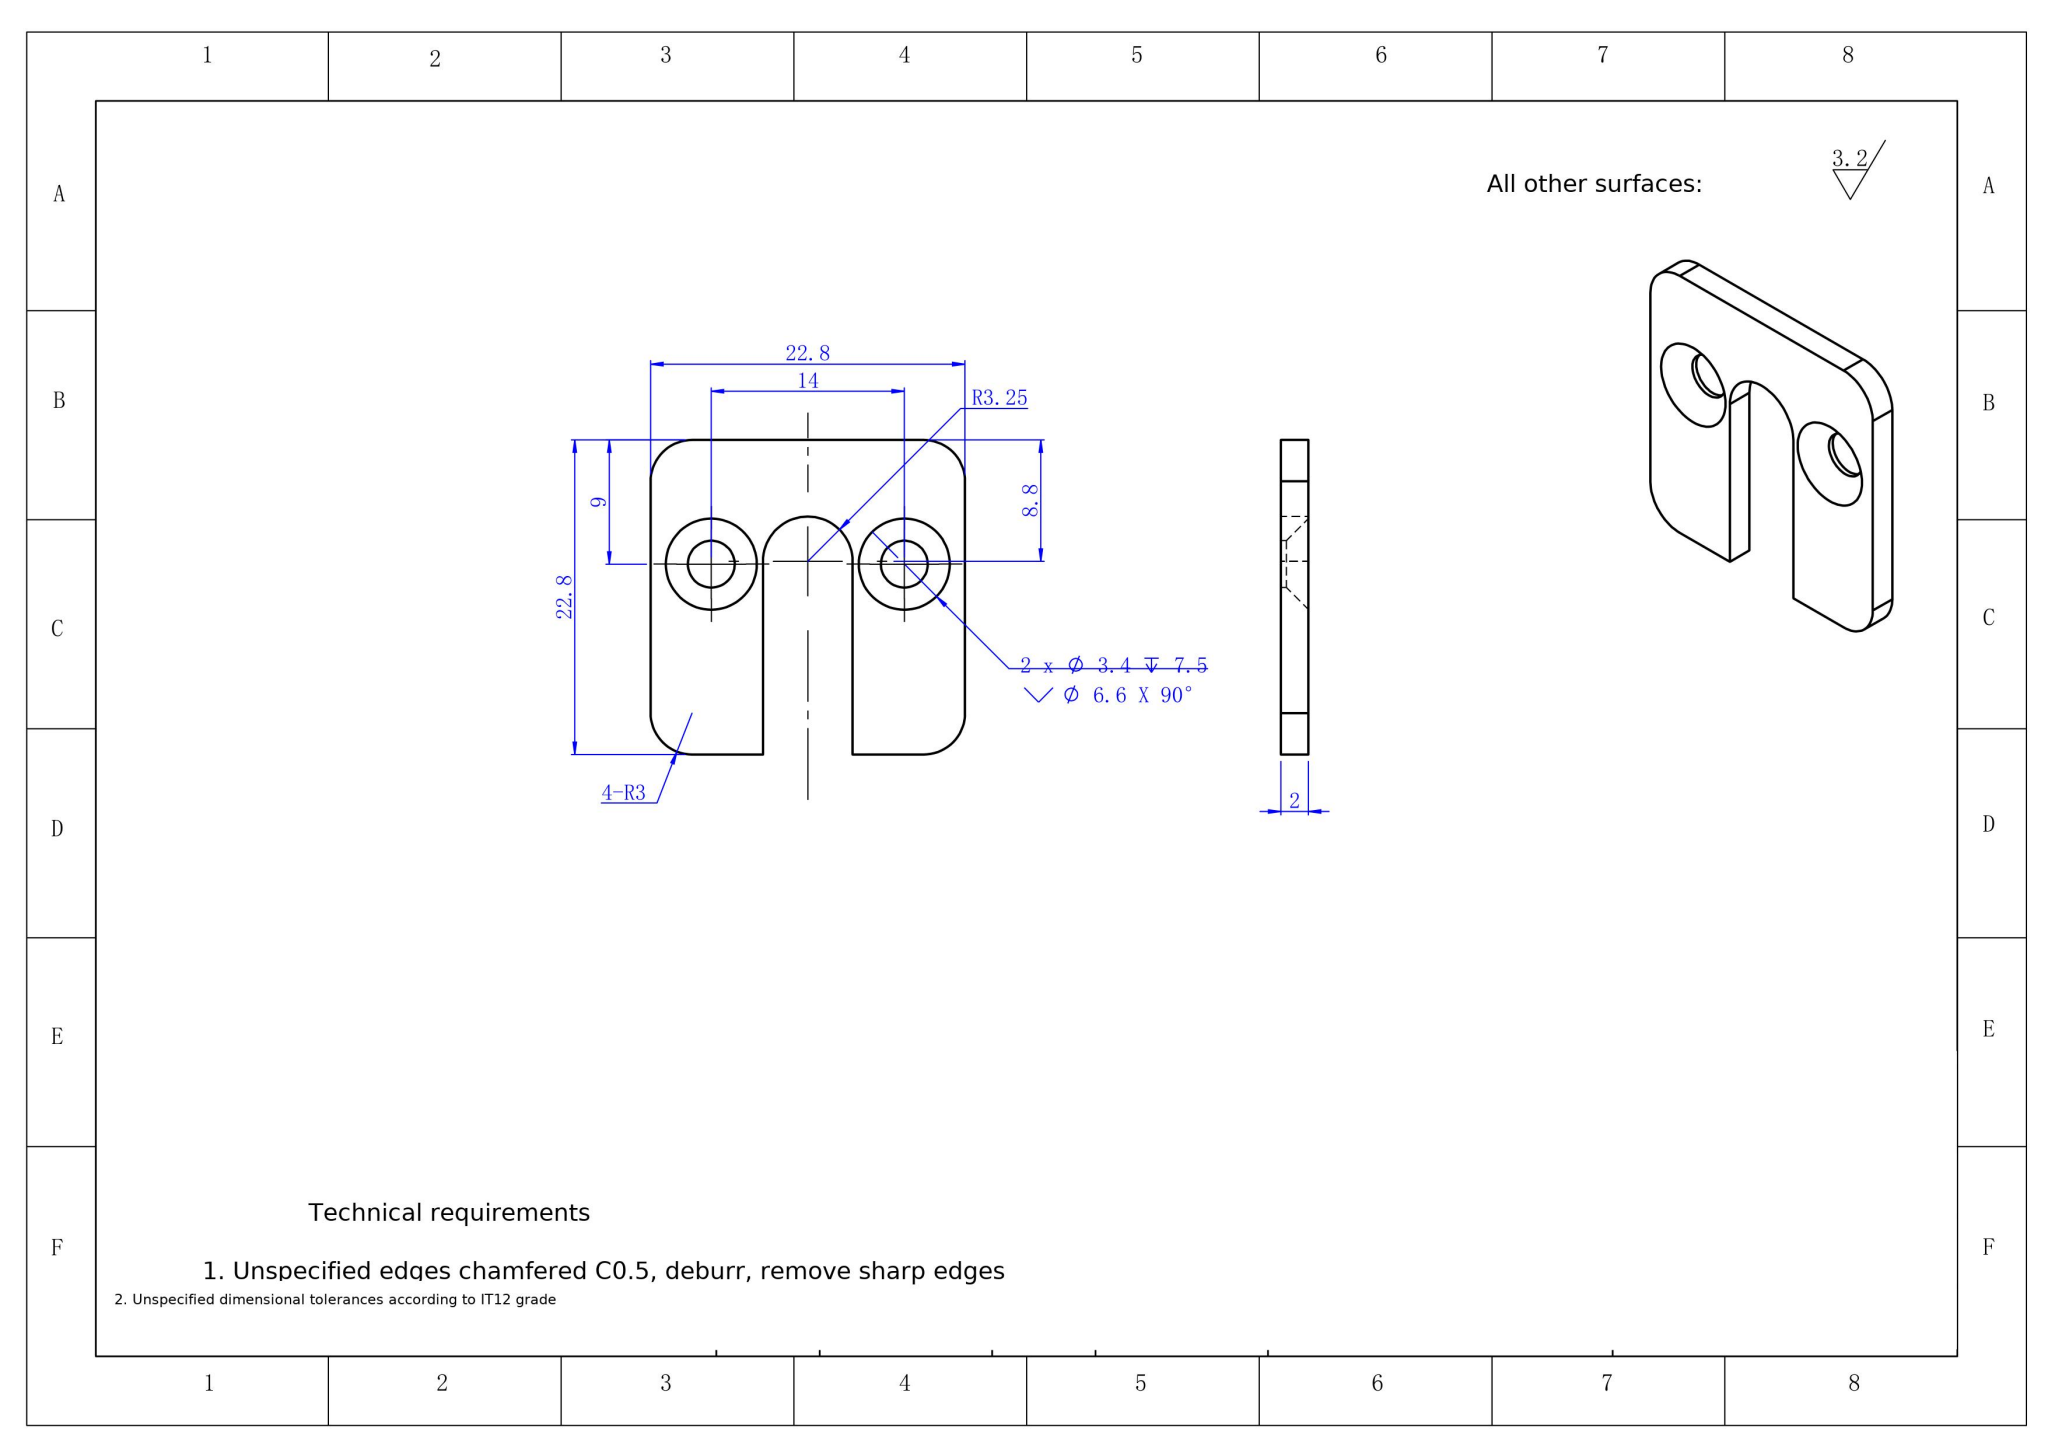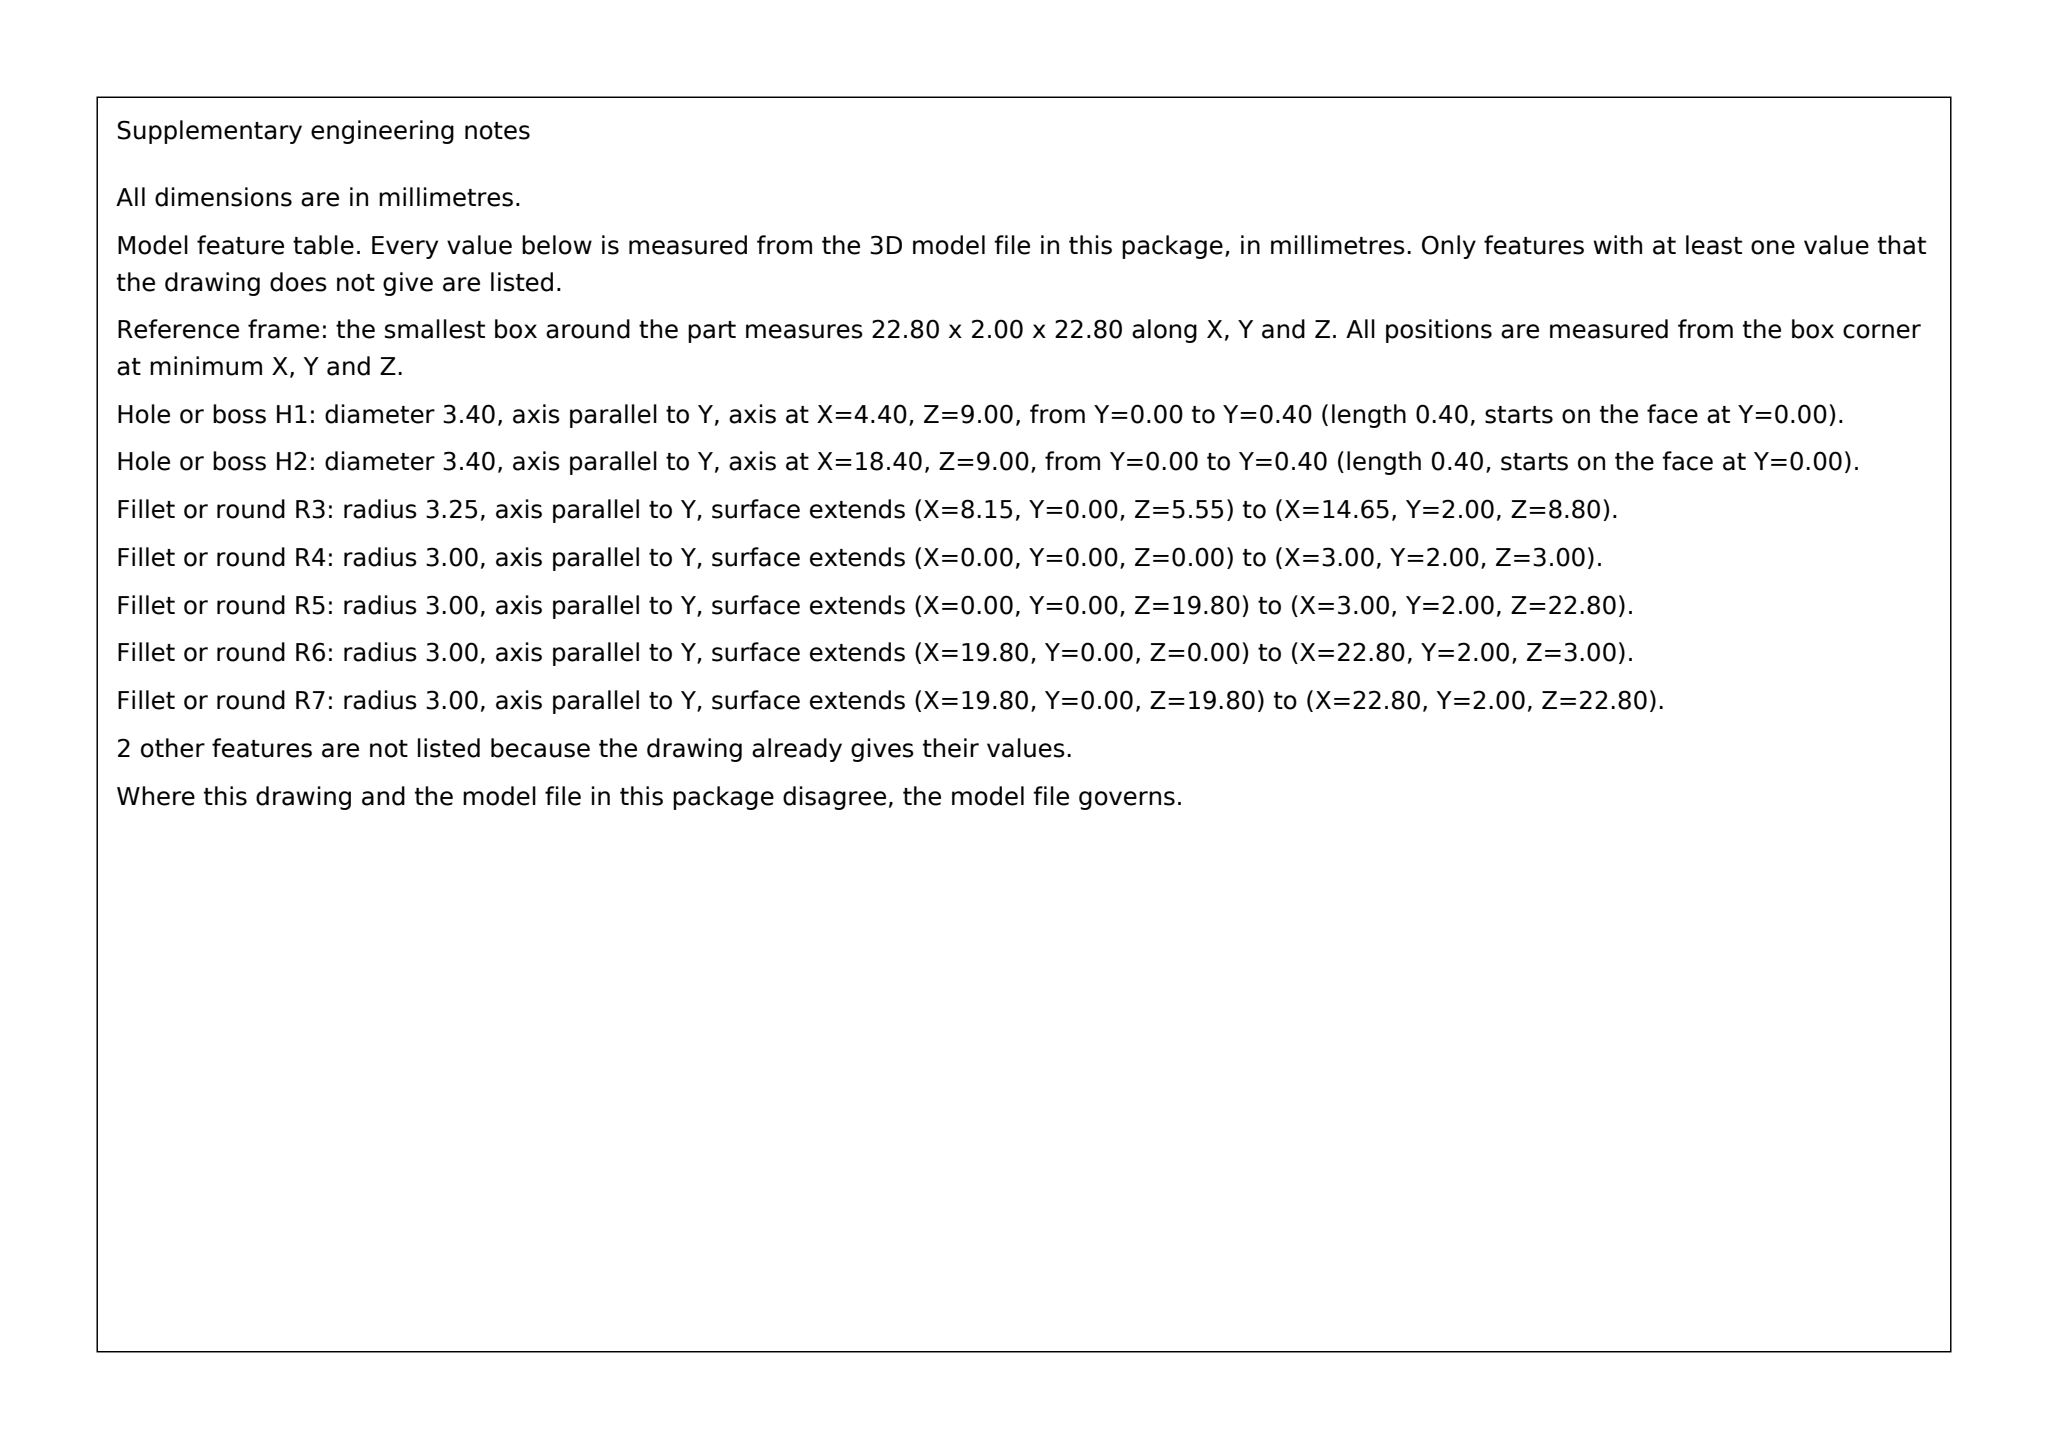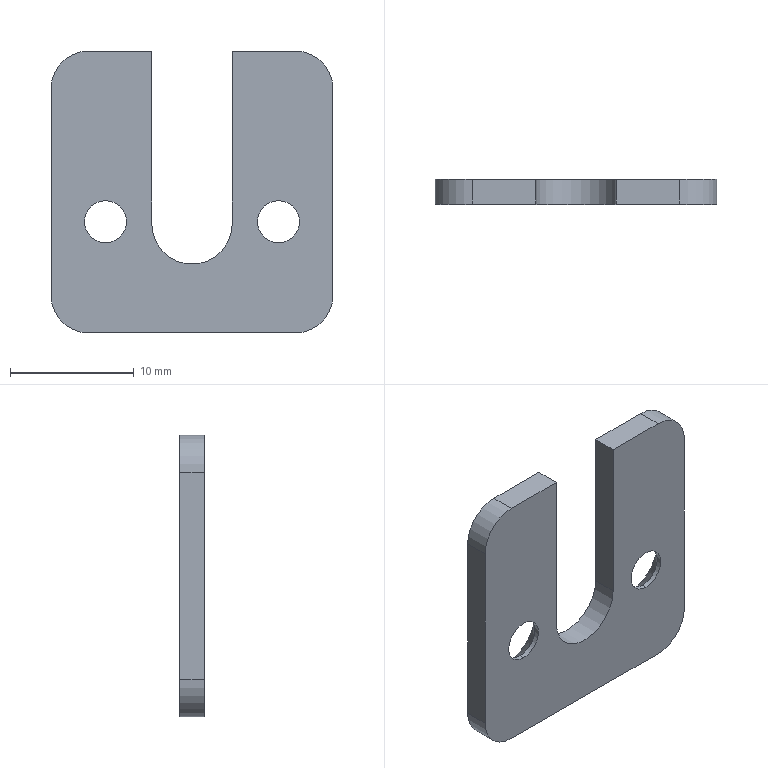Part | SolidWorks | mm | 1 solid | 22 faces | box 22.8 x 2 x 22.8 mm | volume 737 mm3 | cylinder 9 | plane 9 | cone 4 | commonest cylinder face diameters 3.4 x4 6 x4 6.5 x1
build123d program:
from build123d import *

# Parameters (mm, degrees)
SKETCH1_W                                         = 22.8
SKETCH1_H                                         = 22.8
BOSS_EXTRUDE1_DEPTH                               = 2
CUT_EXTRUDE1_DEPTH                                = 26.57
HOLE_SIZE_ACCORDING_TO_SLOTTED_COUNTE_D           = 3.4
HOLE_SIZE_ACCORDING_TO_SLOTTED_COUNTE_DEPTH       = 7.5
HOLE_SIZE_ACCORDING_TO_SLOTTED_COUNTE_CSINK_D     = 6.6
HOLE_SIZE_ACCORDING_TO_SLOTTED_COUNTE_CSINK_ANGLE = 90
HOLE_SIZE_ACCORDING_TO_SLOTTED_COUNTE_TIP         = 1.021
FILLET1_R                                         = 3


with BuildPart() as part:
    # Sketch1 → Boss-Extrude1 (new body)
    with BuildSketch(Plane(origin=(0, 0, 0), x_dir=(1, 0, 0), z_dir=(0, 1, 0))):
        with Locations((0, 11.4)):
            Rectangle(SKETCH1_W, SKETCH1_H)
    extrude(amount=BOSS_EXTRUDE1_DEPTH)

    # Sketch2 → Cut-Extrude1 (cut, through all)
    with BuildSketch(Plane(origin=(0, 2, 0), x_dir=(1, 0, 0), z_dir=(0, 1, 0))):
        with BuildLine():
            Line((-3.25, 0), (-3.25, 14))
            ThreePointArc((-3.25, 14), (0, 17.25), (3.25, 14))
            Line((3.25, 14), (3.25, 0))
            ThreePointArc((3.25, 0), (0, -3.25), (-3.25, 0))
        make_face()
    extrude(amount=-CUT_EXTRUDE1_DEPTH, mode=Mode.SUBTRACT)

    # Hole Size _ according to_ Slotted Counte
    with Locations(Plane(origin=(0, 2, 0), x_dir=(1, 0, 0), z_dir=(0, 1, 0))):
        with Locations((-7, 13.8), (7, 13.8)):
            CounterSinkHole(HOLE_SIZE_ACCORDING_TO_SLOTTED_COUNTE_D / 2, HOLE_SIZE_ACCORDING_TO_SLOTTED_COUNTE_CSINK_D / 2, depth=HOLE_SIZE_ACCORDING_TO_SLOTTED_COUNTE_DEPTH, counter_sink_angle=HOLE_SIZE_ACCORDING_TO_SLOTTED_COUNTE_CSINK_ANGLE)
            with Locations((0, 0, -(HOLE_SIZE_ACCORDING_TO_SLOTTED_COUNTE_DEPTH + HOLE_SIZE_ACCORDING_TO_SLOTTED_COUNTE_TIP / 2))):  # 118° drill point
                Cone(0, HOLE_SIZE_ACCORDING_TO_SLOTTED_COUNTE_D / 2, HOLE_SIZE_ACCORDING_TO_SLOTTED_COUNTE_TIP, mode=Mode.SUBTRACT)

    # Fillet1
    fillet1_edges = [part.edges().sort_by_distance(p)[0] for p in [
        (-11.4, 1, -22.8),
        (11.4, 1, -22.8),
        (11.4, 1, 0),
        (-11.4, 1, 0),
    ]]
    fillet(fillet1_edges, radius=FILLET1_R)


solid = part.part
STEP:
#1=CARTESIAN_POINT('',(-7.,0.4,-15.5));
#2=VERTEX_POINT('',#1);
#3=CARTESIAN_POINT('',(-7.,0.4,-12.1));
#4=VERTEX_POINT('',#3);
#5=CARTESIAN_POINT('',(-7.,0.4,-13.8));
#6=DIRECTION('',(0.,1.,0.));
#7=DIRECTION('',(0.,0.,1.));
#8=AXIS2_PLACEMENT_3D('',#5,#6,#7);
#9=CIRCLE('',#8,1.7);
#10=EDGE_CURVE('',#2,#4,#9,.T.);
#11=ORIENTED_EDGE('',*,*,#10,.F.);
#12=CARTESIAN_POINT('',(-7.,2.,-17.1));
#13=VERTEX_POINT('',#12);
#14=CARTESIAN_POINT('',(-7.,2.,-17.1));
#15=DIRECTION('',(0.,0.7071,-0.7071));
#16=VECTOR('',#15,1000.);
#17=LINE('',#14,#16);
#18=EDGE_CURVE('',#2,#13,#17,.T.);
#19=ORIENTED_EDGE('',*,*,#18,.T.);
#20=CARTESIAN_POINT('',(-7.,2.,-10.5));
#21=VERTEX_POINT('',#20);
#22=CARTESIAN_POINT('',(-7.,2.,-13.8));
#23=DIRECTION('',(0.,1.,0.));
#24=DIRECTION('',(0.,0.,1.));
#25=AXIS2_PLACEMENT_3D('',#22,#23,#24);
#26=CIRCLE('',#25,3.3);
#27=EDGE_CURVE('',#13,#21,#26,.T.);
#28=ORIENTED_EDGE('',*,*,#27,.T.);
#29=CARTESIAN_POINT('',(-7.,2.,-10.5));
#30=DIRECTION('',(0.,0.7071,0.7071));
#31=VECTOR('',#30,1000.);
#32=LINE('',#29,#31);
#33=EDGE_CURVE('',#4,#21,#32,.T.);
#34=ORIENTED_EDGE('',*,*,#33,.F.);
#35=EDGE_LOOP('',(#11,#19,#28,#34));
#36=FACE_OUTER_BOUND('',#35,.T.);
#37=CARTESIAN_POINT('',(-7.,2.,-13.8));
#38=DIRECTION('',(0.,1.,0.));
#39=DIRECTION('',(0.,0.,1.));
#40=AXIS2_PLACEMENT_3D('',#37,#38,#39);
#41=CONICAL_SURFACE('',#40,3.3,0.7854);
#42=ADVANCED_FACE('',(#36),#41,.F.);
#43=CARTESIAN_POINT('',(-7.,0.,-12.1));
#44=VERTEX_POINT('',#43);
#45=CARTESIAN_POINT('',(-7.,0.,-15.5));
#46=VERTEX_POINT('',#45);
#47=CARTESIAN_POINT('',(-7.,0.,-13.8));
#48=DIRECTION('',(0.,-1.,0.));
#49=DIRECTION('',(0.,0.,-1.));
#50=AXIS2_PLACEMENT_3D('',#47,#48,#49);
#51=CIRCLE('',#50,1.7);
#52=EDGE_CURVE('',#44,#46,#51,.T.);
#53=ORIENTED_EDGE('',*,*,#52,.T.);
#54=CARTESIAN_POINT('',(-7.,2.,-15.5));
#55=DIRECTION('',(0.,1.,0.));
#56=VECTOR('',#55,1000.);
#57=LINE('',#54,#56);
#58=EDGE_CURVE('',#46,#2,#57,.T.);
#59=ORIENTED_EDGE('',*,*,#58,.T.);
#60=ORIENTED_EDGE('',*,*,#10,.T.);
#61=CARTESIAN_POINT('',(-7.,2.,-12.1));
#62=DIRECTION('',(0.,1.,0.));
#63=VECTOR('',#62,1000.);
#64=LINE('',#61,#63);
#65=EDGE_CURVE('',#44,#4,#64,.T.);
#66=ORIENTED_EDGE('',*,*,#65,.F.);
#67=EDGE_LOOP('',(#53,#59,#60,#66));
#68=FACE_OUTER_BOUND('',#67,.T.);
#69=CARTESIAN_POINT('',(-7.,2.,-13.8));
#70=DIRECTION('',(0.,1.,0.));
#71=DIRECTION('',(0.,0.,1.));
#72=AXIS2_PLACEMENT_3D('',#69,#70,#71);
#73=CYLINDRICAL_SURFACE('',#72,1.7);
#74=ADVANCED_FACE('',(#68),#73,.F.);
#75=CARTESIAN_POINT('',(7.,0.4,-15.5));
#76=VERTEX_POINT('',#75);
#77=CARTESIAN_POINT('',(7.,0.4,-12.1));
#78=VERTEX_POINT('',#77);
#79=CARTESIAN_POINT('',(7.,0.4,-13.8));
#80=DIRECTION('',(0.,1.,0.));
#81=DIRECTION('',(0.,0.,1.));
#82=AXIS2_PLACEMENT_3D('',#79,#80,#81);
#83=CIRCLE('',#82,1.7);
#84=EDGE_CURVE('',#76,#78,#83,.T.);
#85=ORIENTED_EDGE('',*,*,#84,.F.);
#86=CARTESIAN_POINT('',(7.,2.,-17.1));
#87=VERTEX_POINT('',#86);
#88=CARTESIAN_POINT('',(7.,2.,-17.1));
#89=DIRECTION('',(0.,0.7071,-0.7071));
#90=VECTOR('',#89,1000.);
#91=LINE('',#88,#90);
#92=EDGE_CURVE('',#76,#87,#91,.T.);
#93=ORIENTED_EDGE('',*,*,#92,.T.);
#94=CARTESIAN_POINT('',(7.,2.,-10.5));
#95=VERTEX_POINT('',#94);
#96=CARTESIAN_POINT('',(7.,2.,-13.8));
#97=DIRECTION('',(0.,1.,0.));
#98=DIRECTION('',(0.,0.,1.));
#99=AXIS2_PLACEMENT_3D('',#96,#97,#98);
#100=CIRCLE('',#99,3.3);
#101=EDGE_CURVE('',#87,#95,#100,.T.);
#102=ORIENTED_EDGE('',*,*,#101,.T.);
#103=CARTESIAN_POINT('',(7.,2.,-10.5));
#104=DIRECTION('',(0.,0.7071,0.7071));
#105=VECTOR('',#104,1000.);
#106=LINE('',#103,#105);
#107=EDGE_CURVE('',#78,#95,#106,.T.);
#108=ORIENTED_EDGE('',*,*,#107,.F.);
#109=EDGE_LOOP('',(#85,#93,#102,#108));
#110=FACE_OUTER_BOUND('',#109,.T.);
#111=CARTESIAN_POINT('',(7.,2.,-13.8));
#112=DIRECTION('',(0.,1.,0.));
#113=DIRECTION('',(0.,0.,1.));
#114=AXIS2_PLACEMENT_3D('',#111,#112,#113);
#115=CONICAL_SURFACE('',#114,3.3,0.7854);
#116=ADVANCED_FACE('',(#110),#115,.F.);
#117=CARTESIAN_POINT('',(7.,0.,-12.1));
#118=VERTEX_POINT('',#117);
#119=CARTESIAN_POINT('',(7.,0.,-15.5));
#120=VERTEX_POINT('',#119);
#121=CARTESIAN_POINT('',(7.,0.,-13.8));
#122=DIRECTION('',(0.,-1.,0.));
#123=DIRECTION('',(0.,0.,-1.));
#124=AXIS2_PLACEMENT_3D('',#121,#122,#123);
#125=CIRCLE('',#124,1.7);
#126=EDGE_CURVE('',#118,#120,#125,.T.);
#127=ORIENTED_EDGE('',*,*,#126,.T.);
#128=CARTESIAN_POINT('',(7.,2.,-15.5));
#129=DIRECTION('',(0.,1.,0.));
#130=VECTOR('',#129,1000.);
#131=LINE('',#128,#130);
#132=EDGE_CURVE('',#120,#76,#131,.T.);
#133=ORIENTED_EDGE('',*,*,#132,.T.);
#134=ORIENTED_EDGE('',*,*,#84,.T.);
#135=CARTESIAN_POINT('',(7.,2.,-12.1));
#136=DIRECTION('',(0.,1.,0.));
#137=VECTOR('',#136,1000.);
#138=LINE('',#135,#137);
#139=EDGE_CURVE('',#118,#78,#138,.T.);
#140=ORIENTED_EDGE('',*,*,#139,.F.);
#141=EDGE_LOOP('',(#127,#133,#134,#140));
#142=FACE_OUTER_BOUND('',#141,.T.);
#143=CARTESIAN_POINT('',(7.,2.,-13.8));
#144=DIRECTION('',(0.,1.,0.));
#145=DIRECTION('',(0.,0.,1.));
#146=AXIS2_PLACEMENT_3D('',#143,#144,#145);
#147=CYLINDRICAL_SURFACE('',#146,1.7);
#148=ADVANCED_FACE('',(#142),#147,.F.);
#149=CARTESIAN_POINT('',(-8.4,2.,0.));
#150=VERTEX_POINT('',#149);
#151=CARTESIAN_POINT('',(-3.25,2.,0.));
#152=VERTEX_POINT('',#151);
#153=CARTESIAN_POINT('',(-11.4,2.,0.));
#154=DIRECTION('',(1.,0.,0.));
#155=VECTOR('',#154,1000.);
#156=LINE('',#153,#155);
#157=EDGE_CURVE('',#150,#152,#156,.T.);
#158=ORIENTED_EDGE('',*,*,#157,.F.);
#159=CARTESIAN_POINT('',(-8.4,0.,0.));
#160=VERTEX_POINT('',#159);
#161=CARTESIAN_POINT('',(-8.4,2.,0.));
#162=DIRECTION('',(0.,-1.,0.));
#163=VECTOR('',#162,1000.);
#164=LINE('',#161,#163);
#165=EDGE_CURVE('',#150,#160,#164,.T.);
#166=ORIENTED_EDGE('',*,*,#165,.T.);
#167=CARTESIAN_POINT('',(-3.25,0.,0.));
#168=VERTEX_POINT('',#167);
#169=CARTESIAN_POINT('',(-11.4,0.,0.));
#170=DIRECTION('',(1.,0.,0.));
#171=VECTOR('',#170,1000.);
#172=LINE('',#169,#171);
#173=EDGE_CURVE('',#160,#168,#172,.T.);
#174=ORIENTED_EDGE('',*,*,#173,.T.);
#175=CARTESIAN_POINT('',(-3.25,0.,0.));
#176=DIRECTION('',(0.,1.,0.));
#177=VECTOR('',#176,1000.);
#178=LINE('',#175,#177);
#179=EDGE_CURVE('',#168,#152,#178,.T.);
#180=ORIENTED_EDGE('',*,*,#179,.T.);
#181=EDGE_LOOP('',(#158,#166,#174,#180));
#182=FACE_OUTER_BOUND('',#181,.T.);
#183=CARTESIAN_POINT('',(-11.4,2.,0.));
#184=DIRECTION('',(0.,0.,-1.));
#185=DIRECTION('',(-1.,0.,0.));
#186=AXIS2_PLACEMENT_3D('',#183,#184,#185);
#187=PLANE('',#186);
#188=ADVANCED_FACE('',(#182),#187,.F.);
#189=CARTESIAN_POINT('',(-11.4,0.,-19.8));
#190=VERTEX_POINT('',#189);
#191=CARTESIAN_POINT('',(-11.4,0.,-3.));
#192=VERTEX_POINT('',#191);
#193=CARTESIAN_POINT('',(-11.4,0.,0.));
#194=DIRECTION('',(0.,0.,1.));
#195=VECTOR('',#194,1000.);
#196=LINE('',#193,#195);
#197=EDGE_CURVE('',#190,#192,#196,.T.);
#198=ORIENTED_EDGE('',*,*,#197,.T.);
#199=CARTESIAN_POINT('',(-11.4,2.,-3.));
#200=VERTEX_POINT('',#199);
#201=CARTESIAN_POINT('',(-11.4,2.,-3.));
#202=DIRECTION('',(0.,1.,0.));
#203=VECTOR('',#202,1000.);
#204=LINE('',#201,#203);
#205=EDGE_CURVE('',#192,#200,#204,.T.);
#206=ORIENTED_EDGE('',*,*,#205,.T.);
#207=CARTESIAN_POINT('',(-11.4,2.,-19.8));
#208=VERTEX_POINT('',#207);
#209=CARTESIAN_POINT('',(-11.4,2.,0.));
#210=DIRECTION('',(0.,0.,1.));
#211=VECTOR('',#210,1000.);
#212=LINE('',#209,#211);
#213=EDGE_CURVE('',#208,#200,#212,.T.);
#214=ORIENTED_EDGE('',*,*,#213,.F.);
#215=CARTESIAN_POINT('',(-11.4,2.,-19.8));
#216=DIRECTION('',(0.,-1.,0.));
#217=VECTOR('',#216,1000.);
#218=LINE('',#215,#217);
#219=EDGE_CURVE('',#208,#190,#218,.T.);
#220=ORIENTED_EDGE('',*,*,#219,.T.);
#221=EDGE_LOOP('',(#198,#206,#214,#220));
#222=FACE_OUTER_BOUND('',#221,.T.);
#223=CARTESIAN_POINT('',(-11.4,2.,0.));
#224=DIRECTION('',(1.,0.,0.));
#225=DIRECTION('',(0.,0.,-1.));
#226=AXIS2_PLACEMENT_3D('',#223,#224,#225);
#227=PLANE('',#226);
#228=ADVANCED_FACE('',(#222),#227,.F.);
#229=CARTESIAN_POINT('',(3.25,0.,0.));
#230=VERTEX_POINT('',#229);
#231=CARTESIAN_POINT('',(8.4,0.,0.));
#232=VERTEX_POINT('',#231);
#233=CARTESIAN_POINT('',(-11.4,0.,0.));
#234=DIRECTION('',(1.,0.,0.));
#235=VECTOR('',#234,1000.);
#236=LINE('',#233,#235);
#237=EDGE_CURVE('',#230,#232,#236,.T.);
#238=ORIENTED_EDGE('',*,*,#237,.T.);
#239=CARTESIAN_POINT('',(8.4,2.,0.));
#240=VERTEX_POINT('',#239);
#241=CARTESIAN_POINT('',(8.4,2.,0.));
#242=DIRECTION('',(0.,1.,0.));
#243=VECTOR('',#242,1000.);
#244=LINE('',#241,#243);
#245=EDGE_CURVE('',#232,#240,#244,.T.);
#246=ORIENTED_EDGE('',*,*,#245,.T.);
#247=CARTESIAN_POINT('',(3.25,2.,0.));
#248=VERTEX_POINT('',#247);
#249=CARTESIAN_POINT('',(-11.4,2.,0.));
#250=DIRECTION('',(1.,0.,0.));
#251=VECTOR('',#250,1000.);
#252=LINE('',#249,#251);
#253=EDGE_CURVE('',#248,#240,#252,.T.);
#254=ORIENTED_EDGE('',*,*,#253,.F.);
#255=CARTESIAN_POINT('',(3.25,0.,0.));
#256=DIRECTION('',(0.,1.,0.));
#257=VECTOR('',#256,1000.);
#258=LINE('',#255,#257);
#259=EDGE_CURVE('',#230,#248,#258,.T.);
#260=ORIENTED_EDGE('',*,*,#259,.F.);
#261=EDGE_LOOP('',(#238,#246,#254,#260));
#262=FACE_OUTER_BOUND('',#261,.T.);
#263=CARTESIAN_POINT('',(-11.4,2.,0.));
#264=DIRECTION('',(0.,0.,-1.));
#265=DIRECTION('',(-1.,0.,0.));
#266=AXIS2_PLACEMENT_3D('',#263,#264,#265);
#267=PLANE('',#266);
#268=ADVANCED_FACE('',(#262),#267,.F.);
#269=CARTESIAN_POINT('',(11.4,2.,-3.));
#270=VERTEX_POINT('',#269);
#271=CARTESIAN_POINT('',(11.4,2.,-19.8));
#272=VERTEX_POINT('',#271);
#273=CARTESIAN_POINT('',(11.4,2.,0.));
#274=DIRECTION('',(0.,0.,-1.));
#275=VECTOR('',#274,1000.);
#276=LINE('',#273,#275);
#277=EDGE_CURVE('',#270,#272,#276,.T.);
#278=ORIENTED_EDGE('',*,*,#277,.F.);
#279=CARTESIAN_POINT('',(11.4,0.,-3.));
#280=VERTEX_POINT('',#279);
#281=CARTESIAN_POINT('',(11.4,2.,-3.));
#282=DIRECTION('',(0.,-1.,0.));
#283=VECTOR('',#282,1000.);
#284=LINE('',#281,#283);
#285=EDGE_CURVE('',#270,#280,#284,.T.);
#286=ORIENTED_EDGE('',*,*,#285,.T.);
#287=CARTESIAN_POINT('',(11.4,0.,-19.8));
#288=VERTEX_POINT('',#287);
#289=CARTESIAN_POINT('',(11.4,0.,0.));
#290=DIRECTION('',(0.,0.,-1.));
#291=VECTOR('',#290,1000.);
#292=LINE('',#289,#291);
#293=EDGE_CURVE('',#280,#288,#292,.T.);
#294=ORIENTED_EDGE('',*,*,#293,.T.);
#295=CARTESIAN_POINT('',(11.4,2.,-19.8));
#296=DIRECTION('',(0.,1.,0.));
#297=VECTOR('',#296,1000.);
#298=LINE('',#295,#297);
#299=EDGE_CURVE('',#288,#272,#298,.T.);
#300=ORIENTED_EDGE('',*,*,#299,.T.);
#301=EDGE_LOOP('',(#278,#286,#294,#300));
#302=FACE_OUTER_BOUND('',#301,.T.);
#303=CARTESIAN_POINT('',(11.4,2.,0.));
#304=DIRECTION('',(-1.,0.,0.));
#305=DIRECTION('',(0.,0.,1.));
#306=AXIS2_PLACEMENT_3D('',#303,#304,#305);
#307=PLANE('',#306);
#308=ADVANCED_FACE('',(#302),#307,.F.);
#309=CARTESIAN_POINT('',(8.4,2.,-22.8));
#310=VERTEX_POINT('',#309);
#311=CARTESIAN_POINT('',(-8.4,2.,-22.8));
#312=VERTEX_POINT('',#311);
#313=CARTESIAN_POINT('',(-11.4,2.,-22.8));
#314=DIRECTION('',(-1.,0.,0.));
#315=VECTOR('',#314,1000.);
#316=LINE('',#313,#315);
#317=EDGE_CURVE('',#310,#312,#316,.T.);
#318=ORIENTED_EDGE('',*,*,#317,.F.);
#319=CARTESIAN_POINT('',(8.4,0.,-22.8));
#320=VERTEX_POINT('',#319);
#321=CARTESIAN_POINT('',(8.4,2.,-22.8));
#322=DIRECTION('',(0.,-1.,0.));
#323=VECTOR('',#322,1000.);
#324=LINE('',#321,#323);
#325=EDGE_CURVE('',#310,#320,#324,.T.);
#326=ORIENTED_EDGE('',*,*,#325,.T.);
#327=CARTESIAN_POINT('',(-8.4,0.,-22.8));
#328=VERTEX_POINT('',#327);
#329=CARTESIAN_POINT('',(-11.4,0.,-22.8));
#330=DIRECTION('',(-1.,0.,0.));
#331=VECTOR('',#330,1000.);
#332=LINE('',#329,#331);
#333=EDGE_CURVE('',#320,#328,#332,.T.);
#334=ORIENTED_EDGE('',*,*,#333,.T.);
#335=CARTESIAN_POINT('',(-8.4,2.,-22.8));
#336=DIRECTION('',(0.,1.,0.));
#337=VECTOR('',#336,1000.);
#338=LINE('',#335,#337);
#339=EDGE_CURVE('',#328,#312,#338,.T.);
#340=ORIENTED_EDGE('',*,*,#339,.T.);
#341=EDGE_LOOP('',(#318,#326,#334,#340));
#342=FACE_OUTER_BOUND('',#341,.T.);
#343=CARTESIAN_POINT('',(-11.4,2.,-22.8));
#344=DIRECTION('',(0.,0.,1.));
#345=DIRECTION('',(1.,0.,0.));
#346=AXIS2_PLACEMENT_3D('',#343,#344,#345);
#347=PLANE('',#346);
#348=ADVANCED_FACE('',(#342),#347,.F.);
#349=CARTESIAN_POINT('',(-7.,2.,-13.8));
#350=DIRECTION('',(0.,1.,0.));
#351=DIRECTION('',(0.,0.,1.));
#352=AXIS2_PLACEMENT_3D('',#349,#350,#351);
#353=CIRCLE('',#352,3.3);
#354=EDGE_CURVE('',#21,#13,#353,.T.);
#355=ORIENTED_EDGE('',*,*,#354,.F.);
#356=ORIENTED_EDGE('',*,*,#27,.F.);
#357=EDGE_LOOP('',(#355,#356));
#358=FACE_BOUND('',#357,.T.);
#359=CARTESIAN_POINT('',(7.,2.,-13.8));
#360=DIRECTION('',(0.,1.,0.));
#361=DIRECTION('',(0.,0.,1.));
#362=AXIS2_PLACEMENT_3D('',#359,#360,#361);
#363=CIRCLE('',#362,3.3);
#364=EDGE_CURVE('',#95,#87,#363,.T.);
#365=ORIENTED_EDGE('',*,*,#364,.F.);
#366=ORIENTED_EDGE('',*,*,#101,.F.);
#367=EDGE_LOOP('',(#365,#366));
#368=FACE_BOUND('',#367,.T.);
#369=ORIENTED_EDGE('',*,*,#213,.T.);
#370=CARTESIAN_POINT('',(-8.4,2.,-3.));
#371=DIRECTION('',(0.,1.,0.));
#372=DIRECTION('',(0.,0.,-1.));
#373=AXIS2_PLACEMENT_3D('',#370,#371,#372);
#374=CIRCLE('',#373,3.);
#375=EDGE_CURVE('',#200,#150,#374,.T.);
#376=ORIENTED_EDGE('',*,*,#375,.T.);
#377=ORIENTED_EDGE('',*,*,#157,.T.);
#378=CARTESIAN_POINT('',(-3.25,2.,-14.));
#379=VERTEX_POINT('',#378);
#380=CARTESIAN_POINT('',(-3.25,2.,0.));
#381=DIRECTION('',(0.,0.,1.));
#382=VECTOR('',#381,1000.);
#383=LINE('',#380,#382);
#384=EDGE_CURVE('',#379,#152,#383,.T.);
#385=ORIENTED_EDGE('',*,*,#384,.F.);
#386=CARTESIAN_POINT('',(3.25,2.,-14.));
#387=VERTEX_POINT('',#386);
#388=CARTESIAN_POINT('',(0.,2.,-14.));
#389=DIRECTION('',(0.,1.,0.));
#390=DIRECTION('',(0.,0.,1.));
#391=AXIS2_PLACEMENT_3D('',#388,#389,#390);
#392=CIRCLE('',#391,3.25);
#393=EDGE_CURVE('',#387,#379,#392,.T.);
#394=ORIENTED_EDGE('',*,*,#393,.F.);
#395=CARTESIAN_POINT('',(3.25,2.,0.));
#396=DIRECTION('',(0.,0.,-1.));
#397=VECTOR('',#396,1000.);
#398=LINE('',#395,#397);
#399=EDGE_CURVE('',#248,#387,#398,.T.);
#400=ORIENTED_EDGE('',*,*,#399,.F.);
#401=ORIENTED_EDGE('',*,*,#253,.T.);
#402=CARTESIAN_POINT('',(8.4,2.,-3.));
#403=DIRECTION('',(0.,1.,0.));
#404=DIRECTION('',(0.,0.,-1.));
#405=AXIS2_PLACEMENT_3D('',#402,#403,#404);
#406=CIRCLE('',#405,3.);
#407=EDGE_CURVE('',#240,#270,#406,.T.);
#408=ORIENTED_EDGE('',*,*,#407,.T.);
#409=ORIENTED_EDGE('',*,*,#277,.T.);
#410=CARTESIAN_POINT('',(8.4,2.,-19.8));
#411=DIRECTION('',(0.,1.,0.));
#412=DIRECTION('',(0.,0.,-1.));
#413=AXIS2_PLACEMENT_3D('',#410,#411,#412);
#414=CIRCLE('',#413,3.);
#415=EDGE_CURVE('',#272,#310,#414,.T.);
#416=ORIENTED_EDGE('',*,*,#415,.T.);
#417=ORIENTED_EDGE('',*,*,#317,.T.);
#418=CARTESIAN_POINT('',(-8.4,2.,-19.8));
#419=DIRECTION('',(0.,1.,0.));
#420=DIRECTION('',(0.,0.,-1.));
#421=AXIS2_PLACEMENT_3D('',#418,#419,#420);
#422=CIRCLE('',#421,3.);
#423=EDGE_CURVE('',#312,#208,#422,.T.);
#424=ORIENTED_EDGE('',*,*,#423,.T.);
#425=EDGE_LOOP('',(#369,#376,#377,#385,#394,#400,#401,#408,#409,#416,#417,#424));
#426=FACE_OUTER_BOUND('',#425,.T.);
#427=CARTESIAN_POINT('',(0.,2.,0.));
#428=DIRECTION('',(0.,-1.,0.));
#429=DIRECTION('',(0.,0.,-1.));
#430=AXIS2_PLACEMENT_3D('',#427,#428,#429);
#431=PLANE('',#430);
#432=ADVANCED_FACE('',(#358,#368,#426),#431,.F.);
#433=ORIENTED_EDGE('',*,*,#52,.F.);
#434=CARTESIAN_POINT('',(-7.,0.,-13.8));
#435=DIRECTION('',(0.,-1.,0.));
#436=DIRECTION('',(0.,0.,-1.));
#437=AXIS2_PLACEMENT_3D('',#434,#435,#436);
#438=CIRCLE('',#437,1.7);
#439=EDGE_CURVE('',#46,#44,#438,.T.);
#440=ORIENTED_EDGE('',*,*,#439,.F.);
#441=EDGE_LOOP('',(#433,#440));
#442=FACE_BOUND('',#441,.T.);
#443=ORIENTED_EDGE('',*,*,#126,.F.);
#444=CARTESIAN_POINT('',(7.,0.,-13.8));
#445=DIRECTION('',(0.,-1.,0.));
#446=DIRECTION('',(0.,0.,-1.));
#447=AXIS2_PLACEMENT_3D('',#444,#445,#446);
#448=CIRCLE('',#447,1.7);
#449=EDGE_CURVE('',#120,#118,#448,.T.);
#450=ORIENTED_EDGE('',*,*,#449,.F.);
#451=EDGE_LOOP('',(#443,#450));
#452=FACE_BOUND('',#451,.T.);
#453=ORIENTED_EDGE('',*,*,#173,.F.);
#454=CARTESIAN_POINT('',(-8.4,0.,-3.));
#455=DIRECTION('',(0.,-1.,0.));
#456=DIRECTION('',(0.,0.,-1.));
#457=AXIS2_PLACEMENT_3D('',#454,#455,#456);
#458=CIRCLE('',#457,3.);
#459=EDGE_CURVE('',#160,#192,#458,.T.);
#460=ORIENTED_EDGE('',*,*,#459,.T.);
#461=ORIENTED_EDGE('',*,*,#197,.F.);
#462=CARTESIAN_POINT('',(-8.4,0.,-19.8));
#463=DIRECTION('',(0.,-1.,0.));
#464=DIRECTION('',(0.,0.,-1.));
#465=AXIS2_PLACEMENT_3D('',#462,#463,#464);
#466=CIRCLE('',#465,3.);
#467=EDGE_CURVE('',#190,#328,#466,.T.);
#468=ORIENTED_EDGE('',*,*,#467,.T.);
#469=ORIENTED_EDGE('',*,*,#333,.F.);
#470=CARTESIAN_POINT('',(8.4,0.,-19.8));
#471=DIRECTION('',(0.,-1.,0.));
#472=DIRECTION('',(0.,0.,-1.));
#473=AXIS2_PLACEMENT_3D('',#470,#471,#472);
#474=CIRCLE('',#473,3.);
#475=EDGE_CURVE('',#320,#288,#474,.T.);
#476=ORIENTED_EDGE('',*,*,#475,.T.);
#477=ORIENTED_EDGE('',*,*,#293,.F.);
#478=CARTESIAN_POINT('',(8.4,0.,-3.));
#479=DIRECTION('',(0.,-1.,0.));
#480=DIRECTION('',(0.,0.,-1.));
#481=AXIS2_PLACEMENT_3D('',#478,#479,#480);
#482=CIRCLE('',#481,3.);
#483=EDGE_CURVE('',#280,#232,#482,.T.);
#484=ORIENTED_EDGE('',*,*,#483,.T.);
#485=ORIENTED_EDGE('',*,*,#237,.F.);
#486=CARTESIAN_POINT('',(3.25,0.,-14.));
#487=VERTEX_POINT('',#486);
#488=CARTESIAN_POINT('',(3.25,0.,0.));
#489=DIRECTION('',(0.,0.,-1.));
#490=VECTOR('',#489,1000.);
#491=LINE('',#488,#490);
#492=EDGE_CURVE('',#230,#487,#491,.T.);
#493=ORIENTED_EDGE('',*,*,#492,.T.);
#494=CARTESIAN_POINT('',(-3.25,0.,-14.));
#495=VERTEX_POINT('',#494);
#496=CARTESIAN_POINT('',(0.,0.,-14.));
#497=DIRECTION('',(0.,1.,0.));
#498=DIRECTION('',(0.,0.,1.));
#499=AXIS2_PLACEMENT_3D('',#496,#497,#498);
#500=CIRCLE('',#499,3.25);
#501=EDGE_CURVE('',#487,#495,#500,.T.);
#502=ORIENTED_EDGE('',*,*,#501,.T.);
#503=CARTESIAN_POINT('',(-3.25,0.,0.));
#504=DIRECTION('',(0.,0.,1.));
#505=VECTOR('',#504,1000.);
#506=LINE('',#503,#505);
#507=EDGE_CURVE('',#495,#168,#506,.T.);
#508=ORIENTED_EDGE('',*,*,#507,.T.);
#509=EDGE_LOOP('',(#453,#460,#461,#468,#469,#476,#477,#484,#485,#493,#502,#508));
#510=FACE_OUTER_BOUND('',#509,.T.);
#511=CARTESIAN_POINT('',(0.,0.,0.));
#512=DIRECTION('',(0.,-1.,0.));
#513=DIRECTION('',(0.,0.,-1.));
#514=AXIS2_PLACEMENT_3D('',#511,#512,#513);
#515=PLANE('',#514);
#516=ADVANCED_FACE('',(#442,#452,#510),#515,.T.);
#517=ORIENTED_EDGE('',*,*,#384,.T.);
#518=ORIENTED_EDGE('',*,*,#179,.F.);
#519=ORIENTED_EDGE('',*,*,#507,.F.);
#520=CARTESIAN_POINT('',(-3.25,0.,-14.));
#521=DIRECTION('',(0.,1.,0.));
#522=VECTOR('',#521,1000.);
#523=LINE('',#520,#522);
#524=EDGE_CURVE('',#495,#379,#523,.T.);
#525=ORIENTED_EDGE('',*,*,#524,.T.);
#526=EDGE_LOOP('',(#517,#518,#519,#525));
#527=FACE_OUTER_BOUND('',#526,.T.);
#528=CARTESIAN_POINT('',(-3.25,0.,0.));
#529=DIRECTION('',(-1.,0.,0.));
#530=DIRECTION('',(0.,0.,1.));
#531=AXIS2_PLACEMENT_3D('',#528,#529,#530);
#532=PLANE('',#531);
#533=ADVANCED_FACE('',(#527),#532,.F.);
#534=ORIENTED_EDGE('',*,*,#393,.T.);
#535=ORIENTED_EDGE('',*,*,#524,.F.);
#536=ORIENTED_EDGE('',*,*,#501,.F.);
#537=CARTESIAN_POINT('',(3.25,0.,-14.));
#538=DIRECTION('',(0.,1.,0.));
#539=VECTOR('',#538,1000.);
#540=LINE('',#537,#539);
#541=EDGE_CURVE('',#487,#387,#540,.T.);
#542=ORIENTED_EDGE('',*,*,#541,.T.);
#543=EDGE_LOOP('',(#534,#535,#536,#542));
#544=FACE_OUTER_BOUND('',#543,.T.);
#545=CARTESIAN_POINT('',(0.,0.,-14.));
#546=DIRECTION('',(0.,1.,0.));
#547=DIRECTION('',(0.,0.,1.));
#548=AXIS2_PLACEMENT_3D('',#545,#546,#547);
#549=CYLINDRICAL_SURFACE('',#548,3.25);
#550=ADVANCED_FACE('',(#544),#549,.F.);
#551=ORIENTED_EDGE('',*,*,#399,.T.);
#552=ORIENTED_EDGE('',*,*,#541,.F.);
#553=ORIENTED_EDGE('',*,*,#492,.F.);
#554=ORIENTED_EDGE('',*,*,#259,.T.);
#555=EDGE_LOOP('',(#551,#552,#553,#554));
#556=FACE_OUTER_BOUND('',#555,.T.);
#557=CARTESIAN_POINT('',(3.25,0.,0.));
#558=DIRECTION('',(1.,0.,0.));
#559=DIRECTION('',(0.,0.,-1.));
#560=AXIS2_PLACEMENT_3D('',#557,#558,#559);
#561=PLANE('',#560);
#562=ADVANCED_FACE('',(#556),#561,.F.);
#563=ORIENTED_EDGE('',*,*,#132,.F.);
#564=ORIENTED_EDGE('',*,*,#449,.T.);
#565=ORIENTED_EDGE('',*,*,#139,.T.);
#566=CARTESIAN_POINT('',(7.,0.4,-13.8));
#567=DIRECTION('',(0.,1.,0.));
#568=DIRECTION('',(0.,0.,1.));
#569=AXIS2_PLACEMENT_3D('',#566,#567,#568);
#570=CIRCLE('',#569,1.7);
#571=EDGE_CURVE('',#78,#76,#570,.T.);
#572=ORIENTED_EDGE('',*,*,#571,.T.);
#573=EDGE_LOOP('',(#563,#564,#565,#572));
#574=FACE_OUTER_BOUND('',#573,.T.);
#575=CARTESIAN_POINT('',(7.,2.,-13.8));
#576=DIRECTION('',(0.,1.,0.));
#577=DIRECTION('',(0.,0.,1.));
#578=AXIS2_PLACEMENT_3D('',#575,#576,#577);
#579=CYLINDRICAL_SURFACE('',#578,1.7);
#580=ADVANCED_FACE('',(#574),#579,.F.);
#581=ORIENTED_EDGE('',*,*,#92,.F.);
#582=ORIENTED_EDGE('',*,*,#571,.F.);
#583=ORIENTED_EDGE('',*,*,#107,.T.);
#584=ORIENTED_EDGE('',*,*,#364,.T.);
#585=EDGE_LOOP('',(#581,#582,#583,#584));
#586=FACE_OUTER_BOUND('',#585,.T.);
#587=CARTESIAN_POINT('',(7.,2.,-13.8));
#588=DIRECTION('',(0.,1.,0.));
#589=DIRECTION('',(0.,0.,1.));
#590=AXIS2_PLACEMENT_3D('',#587,#588,#589);
#591=CONICAL_SURFACE('',#590,3.3,0.7854);
#592=ADVANCED_FACE('',(#586),#591,.F.);
#593=ORIENTED_EDGE('',*,*,#58,.F.);
#594=ORIENTED_EDGE('',*,*,#439,.T.);
#595=ORIENTED_EDGE('',*,*,#65,.T.);
#596=CARTESIAN_POINT('',(-7.,0.4,-13.8));
#597=DIRECTION('',(0.,1.,0.));
#598=DIRECTION('',(0.,0.,1.));
#599=AXIS2_PLACEMENT_3D('',#596,#597,#598);
#600=CIRCLE('',#599,1.7);
#601=EDGE_CURVE('',#4,#2,#600,.T.);
#602=ORIENTED_EDGE('',*,*,#601,.T.);
#603=EDGE_LOOP('',(#593,#594,#595,#602));
#604=FACE_OUTER_BOUND('',#603,.T.);
#605=CARTESIAN_POINT('',(-7.,2.,-13.8));
#606=DIRECTION('',(0.,1.,0.));
#607=DIRECTION('',(0.,0.,1.));
#608=AXIS2_PLACEMENT_3D('',#605,#606,#607);
#609=CYLINDRICAL_SURFACE('',#608,1.7);
#610=ADVANCED_FACE('',(#604),#609,.F.);
#611=ORIENTED_EDGE('',*,*,#18,.F.);
#612=ORIENTED_EDGE('',*,*,#601,.F.);
#613=ORIENTED_EDGE('',*,*,#33,.T.);
#614=ORIENTED_EDGE('',*,*,#354,.T.);
#615=EDGE_LOOP('',(#611,#612,#613,#614));
#616=FACE_OUTER_BOUND('',#615,.T.);
#617=CARTESIAN_POINT('',(-7.,2.,-13.8));
#618=DIRECTION('',(0.,1.,0.));
#619=DIRECTION('',(0.,0.,1.));
#620=AXIS2_PLACEMENT_3D('',#617,#618,#619);
#621=CONICAL_SURFACE('',#620,3.3,0.7854);
#622=ADVANCED_FACE('',(#616),#621,.F.);
#623=ORIENTED_EDGE('',*,*,#375,.F.);
#624=ORIENTED_EDGE('',*,*,#205,.F.);
#625=ORIENTED_EDGE('',*,*,#459,.F.);
#626=ORIENTED_EDGE('',*,*,#165,.F.);
#627=EDGE_LOOP('',(#623,#624,#625,#626));
#628=FACE_OUTER_BOUND('',#627,.T.);
#629=CARTESIAN_POINT('',(-8.4,2.,-3.));
#630=DIRECTION('',(0.,-1.,0.));
#631=DIRECTION('',(0.,0.,-1.));
#632=AXIS2_PLACEMENT_3D('',#629,#630,#631);
#633=CYLINDRICAL_SURFACE('',#632,3.);
#634=ADVANCED_FACE('',(#628),#633,.T.);
#635=ORIENTED_EDGE('',*,*,#407,.F.);
#636=ORIENTED_EDGE('',*,*,#245,.F.);
#637=ORIENTED_EDGE('',*,*,#483,.F.);
#638=ORIENTED_EDGE('',*,*,#285,.F.);
#639=EDGE_LOOP('',(#635,#636,#637,#638));
#640=FACE_OUTER_BOUND('',#639,.T.);
#641=CARTESIAN_POINT('',(8.4,2.,-3.));
#642=DIRECTION('',(0.,-1.,0.));
#643=DIRECTION('',(0.,0.,-1.));
#644=AXIS2_PLACEMENT_3D('',#641,#642,#643);
#645=CYLINDRICAL_SURFACE('',#644,3.);
#646=ADVANCED_FACE('',(#640),#645,.T.);
#647=ORIENTED_EDGE('',*,*,#415,.F.);
#648=ORIENTED_EDGE('',*,*,#299,.F.);
#649=ORIENTED_EDGE('',*,*,#475,.F.);
#650=ORIENTED_EDGE('',*,*,#325,.F.);
#651=EDGE_LOOP('',(#647,#648,#649,#650));
#652=FACE_OUTER_BOUND('',#651,.T.);
#653=CARTESIAN_POINT('',(8.4,2.,-19.8));
#654=DIRECTION('',(0.,-1.,0.));
#655=DIRECTION('',(0.,0.,-1.));
#656=AXIS2_PLACEMENT_3D('',#653,#654,#655);
#657=CYLINDRICAL_SURFACE('',#656,3.);
#658=ADVANCED_FACE('',(#652),#657,.T.);
#659=ORIENTED_EDGE('',*,*,#423,.F.);
#660=ORIENTED_EDGE('',*,*,#339,.F.);
#661=ORIENTED_EDGE('',*,*,#467,.F.);
#662=ORIENTED_EDGE('',*,*,#219,.F.);
#663=EDGE_LOOP('',(#659,#660,#661,#662));
#664=FACE_OUTER_BOUND('',#663,.T.);
#665=CARTESIAN_POINT('',(-8.4,2.,-19.8));
#666=DIRECTION('',(0.,-1.,0.));
#667=DIRECTION('',(0.,0.,-1.));
#668=AXIS2_PLACEMENT_3D('',#665,#666,#667);
#669=CYLINDRICAL_SURFACE('',#668,3.);
#670=ADVANCED_FACE('',(#664),#669,.T.);
#671=CLOSED_SHELL('',(#42,#74,#116,#148,#188,#228,#268,#308,#348,#432,#516,#533,#550,#562,#580,#592,#610,#622,#634,#646,#658,#670));
#672=MANIFOLD_SOLID_BREP('',#671);
#673=CARTESIAN_POINT('',(0.,0.,0.));
#674=DIRECTION('',(0.,0.,1.));
#675=DIRECTION('',(1.,0.,0.));
#676=AXIS2_PLACEMENT_3D('',#673,#674,#675);
#677=(LENGTH_UNIT()NAMED_UNIT(*)SI_UNIT(.MILLI.,.METRE.));
#678=UNCERTAINTY_MEASURE_WITH_UNIT(LENGTH_MEASURE(0.00001),#677,'','');
#679=(NAMED_UNIT(*)PLANE_ANGLE_UNIT()SI_UNIT($,.RADIAN.));
#680=(NAMED_UNIT(*)SI_UNIT($,.STERADIAN.)SOLID_ANGLE_UNIT());
#681=(GEOMETRIC_REPRESENTATION_CONTEXT(3)GLOBAL_UNCERTAINTY_ASSIGNED_CONTEXT((#678))GLOBAL_UNIT_ASSIGNED_CONTEXT((#677,#679,#680))REPRESENTATION_CONTEXT('',''));
#682=ADVANCED_BREP_SHAPE_REPRESENTATION('',(#672,#676),#681);